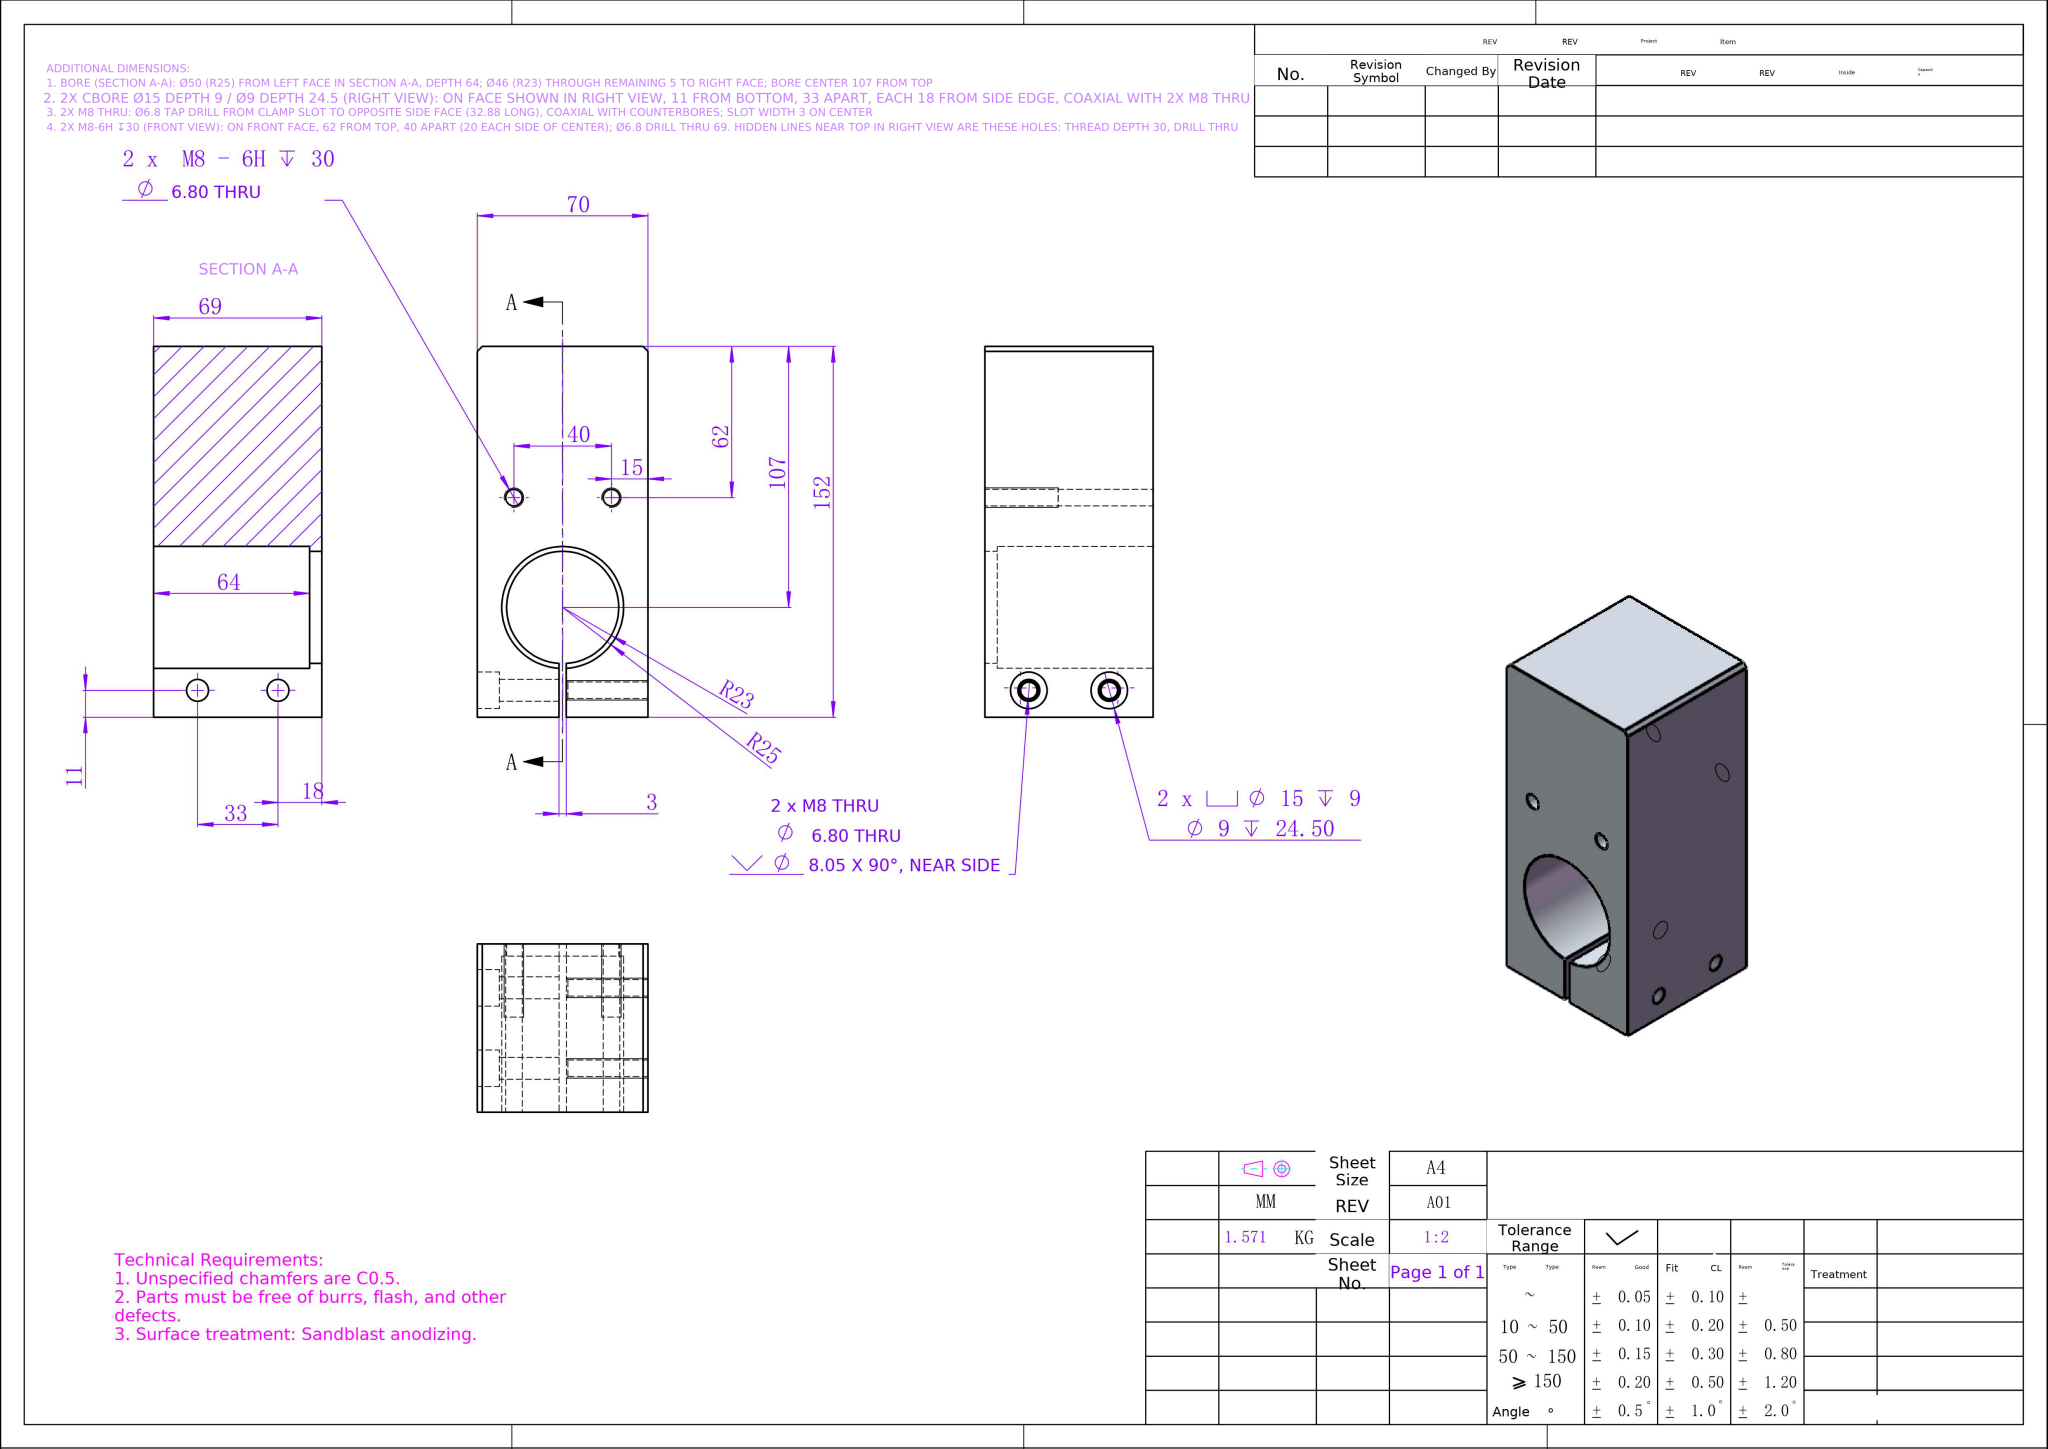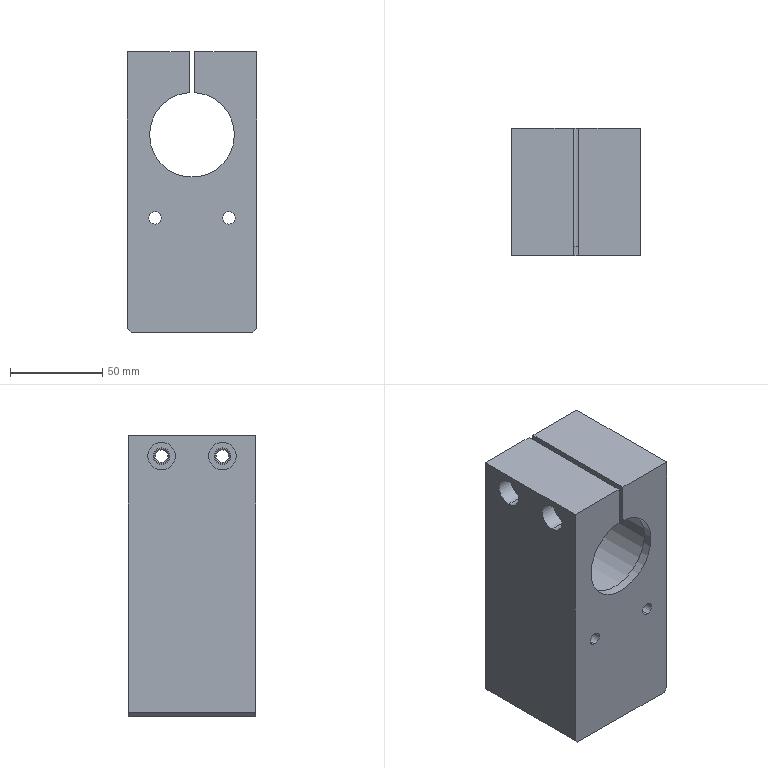Part | NX | mm | 1 solid | 36 faces | box 70 x 69 x 152 mm | volume 581986 mm3 | cylinder 18 | plane 14 | cone 4 | commonest cylinder face diameters 6.8 x8 9 x4 15 x4 50 x1 46 x1